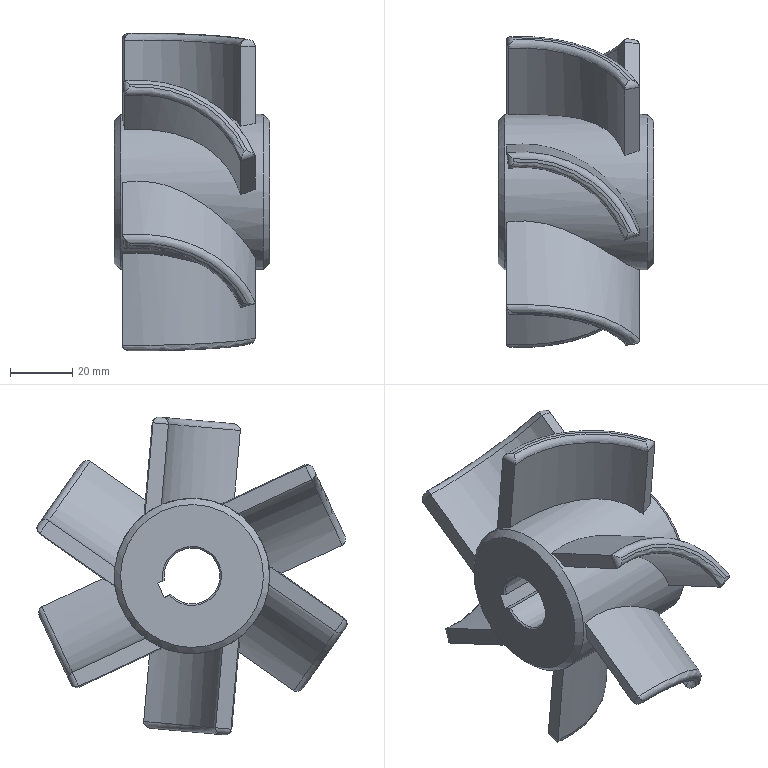Component | NX | FLYWHEEL | 1 solid | 65 faces | volume 125421 mm3 | cylinder 26 | plane 23 | torus 12 | cone 4 | commonest cylinder face diameters 4 x12 79.935 x6 69.935 x6 50 x1 18 x1